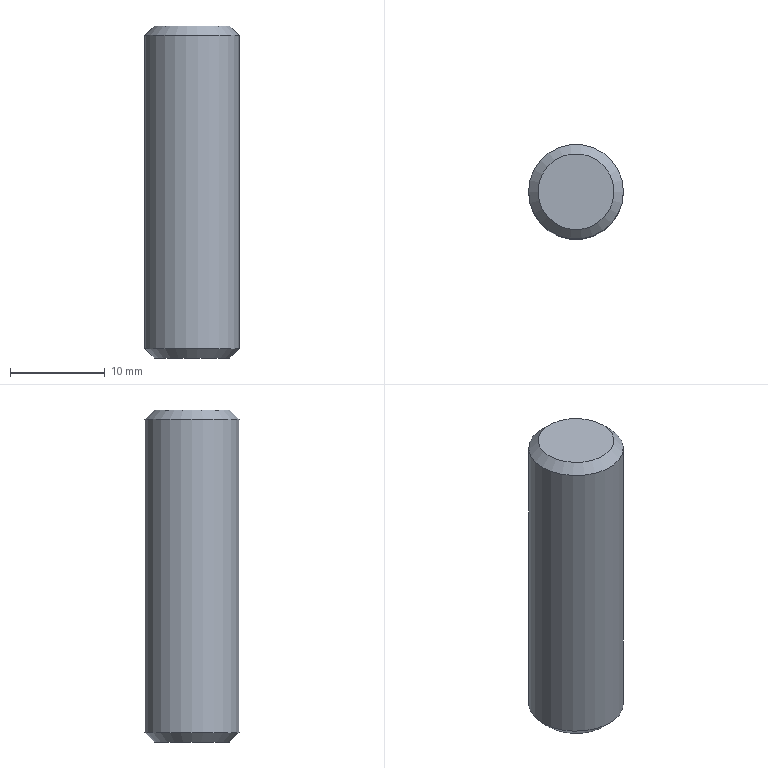Component | NX | EJECTOR_ROD | 1 solid | 5 faces | box 10 x 10 x 35 mm | volume 2720 mm3 | plane 2 | cone 2 | cylinder 1 | commonest cylinder face diameters 10 x1
STEP:
#1=CARTESIAN_POINT('',(0.,0.,0.));
#2=DIRECTION('',(0.,0.,1.));
#3=DIRECTION('',(1.,0.,0.));
#4=AXIS2_PLACEMENT_3D('',#1,#2,#3);
#5=CARTESIAN_POINT('',(24.,80.,198.));
#6=VERTEX_POINT('',#5);
#7=CARTESIAN_POINT('',(20.,80.,198.));
#8=DIRECTION('',(0.,0.,1.));
#9=DIRECTION('',(1.,0.,0.));
#10=AXIS2_PLACEMENT_3D('',#7,#8,#9);
#11=CIRCLE('',#10,4.);
#12=CARTESIAN_POINT('',(20.,80.,198.));
#13=DIRECTION('',(0.,0.,1.));
#14=DIRECTION('',(1.,0.,0.));
#15=AXIS2_PLACEMENT_3D('',#12,#13,#14);
#16=PLANE('',#15);
#17=CARTESIAN_POINT('',(0.,0.));
#18=DIRECTION('',(1.,0.));
#19=AXIS2_PLACEMENT_2D('',#17,#18);
#20=CIRCLE('',#19,4.);
#21=(GEOMETRIC_REPRESENTATION_CONTEXT(2)PARAMETRIC_REPRESENTATION_CONTEXT()REPRESENTATION_CONTEXT('',''));
#22=DEFINITIONAL_REPRESENTATION('',(#20),#21);
#23=PCURVE('',#16,#22);
#24=CARTESIAN_POINT('',(20.,80.,197.));
#25=DIRECTION('',(0.,0.,-1.));
#26=DIRECTION('',(-1.,0.,0.));
#27=AXIS2_PLACEMENT_3D('',#24,#25,#26);
#28=CONICAL_SURFACE('',#27,5.,0.7854);
#29=CARTESIAN_POINT('',(9.425,-1.));
#30=DIRECTION('',(-1.,0.));
#31=VECTOR('',#30,1.);
#32=LINE('',#29,#31);
#33=(GEOMETRIC_REPRESENTATION_CONTEXT(2)PARAMETRIC_REPRESENTATION_CONTEXT()REPRESENTATION_CONTEXT('',''));
#34=DEFINITIONAL_REPRESENTATION('',(#32),#33);
#35=PCURVE('',#28,#34);
#36=SURFACE_CURVE('',#11,(#23,#35),.PCURVE_S1.);
#37=EDGE_CURVE('',#6,#6,#36,.T.);
#38=ORIENTED_EDGE('',*,*,#37,.T.);
#39=EDGE_LOOP('',(#38));
#40=FACE_BOUND('',#39,.T.);
#41=ADVANCED_FACE('',(#40),#16,.T.);
#42=CARTESIAN_POINT('',(16.,80.,163.));
#43=VERTEX_POINT('',#42);
#44=CARTESIAN_POINT('',(20.,80.,163.));
#45=DIRECTION('',(0.,0.,-1.));
#46=DIRECTION('',(-1.,0.,0.));
#47=AXIS2_PLACEMENT_3D('',#44,#45,#46);
#48=CIRCLE('',#47,4.);
#49=CARTESIAN_POINT('',(20.,80.,163.));
#50=DIRECTION('',(0.,0.,-1.));
#51=DIRECTION('',(-1.,0.,0.));
#52=AXIS2_PLACEMENT_3D('',#49,#50,#51);
#53=PLANE('',#52);
#54=CARTESIAN_POINT('',(0.,0.));
#55=DIRECTION('',(1.,0.));
#56=AXIS2_PLACEMENT_2D('',#54,#55);
#57=CIRCLE('',#56,4.);
#58=(GEOMETRIC_REPRESENTATION_CONTEXT(2)PARAMETRIC_REPRESENTATION_CONTEXT()REPRESENTATION_CONTEXT('',''));
#59=DEFINITIONAL_REPRESENTATION('',(#57),#58);
#60=PCURVE('',#53,#59);
#61=CARTESIAN_POINT('',(20.,80.,164.));
#62=DIRECTION('',(0.,0.,1.));
#63=DIRECTION('',(1.,0.,0.));
#64=AXIS2_PLACEMENT_3D('',#61,#62,#63);
#65=CONICAL_SURFACE('',#64,5.,0.7854);
#66=CARTESIAN_POINT('',(9.425,-1.));
#67=DIRECTION('',(-1.,0.));
#68=VECTOR('',#67,1.);
#69=LINE('',#66,#68);
#70=(GEOMETRIC_REPRESENTATION_CONTEXT(2)PARAMETRIC_REPRESENTATION_CONTEXT()REPRESENTATION_CONTEXT('',''));
#71=DEFINITIONAL_REPRESENTATION('',(#69),#70);
#72=PCURVE('',#65,#71);
#73=SURFACE_CURVE('',#48,(#60,#72),.PCURVE_S1.);
#74=EDGE_CURVE('',#43,#43,#73,.T.);
#75=ORIENTED_EDGE('',*,*,#74,.T.);
#76=EDGE_LOOP('',(#75));
#77=FACE_BOUND('',#76,.T.);
#78=ADVANCED_FACE('',(#77),#53,.T.);
#79=CARTESIAN_POINT('',(15.,80.,164.));
#80=VERTEX_POINT('',#79);
#81=CARTESIAN_POINT('',(25.,80.,164.));
#82=VERTEX_POINT('',#81);
#83=CARTESIAN_POINT('',(20.,80.,164.));
#84=DIRECTION('',(0.,0.,1.));
#85=DIRECTION('',(-1.,0.,0.));
#86=AXIS2_PLACEMENT_3D('',#83,#84,#85);
#87=CIRCLE('',#86,5.);
#88=CARTESIAN_POINT('',(20.,80.,163.));
#89=DIRECTION('',(0.,0.,1.));
#90=DIRECTION('',(1.,0.,0.));
#91=AXIS2_PLACEMENT_3D('',#88,#89,#90);
#92=CYLINDRICAL_SURFACE('',#91,5.);
#93=CARTESIAN_POINT('',(3.142,1.));
#94=DIRECTION('',(1.,0.));
#95=VECTOR('',#94,1.);
#96=LINE('',#93,#95);
#97=(GEOMETRIC_REPRESENTATION_CONTEXT(2)PARAMETRIC_REPRESENTATION_CONTEXT()REPRESENTATION_CONTEXT('',''));
#98=DEFINITIONAL_REPRESENTATION('',(#96),#97);
#99=PCURVE('',#92,#98);
#100=CARTESIAN_POINT('',(3.142,0.));
#101=DIRECTION('',(1.,0.));
#102=VECTOR('',#101,1.);
#103=LINE('',#100,#102);
#104=(GEOMETRIC_REPRESENTATION_CONTEXT(2)PARAMETRIC_REPRESENTATION_CONTEXT()REPRESENTATION_CONTEXT('',''));
#105=DEFINITIONAL_REPRESENTATION('',(#103),#104);
#106=PCURVE('',#65,#105);
#107=SURFACE_CURVE('',#87,(#99,#106),.PCURVE_S1.);
#108=EDGE_CURVE('',#80,#82,#107,.T.);
#109=ORIENTED_EDGE('',*,*,#108,.T.);
#110=CARTESIAN_POINT('',(25.,80.,197.));
#111=VERTEX_POINT('',#110);
#112=CARTESIAN_POINT('',(25.,80.,164.));
#113=CARTESIAN_POINT('',(25.,80.,197.));
#114=B_SPLINE_CURVE_WITH_KNOTS('',1,(#112,#113),.UNSPECIFIED.,.F.,.F.,(2,2),(1.,34.),.PIECEWISE_BEZIER_KNOTS.);
#115=CARTESIAN_POINT('',(6.283,0.));
#116=DIRECTION('',(0.,1.));
#117=VECTOR('',#116,1.);
#118=LINE('',#115,#117);
#119=(GEOMETRIC_REPRESENTATION_CONTEXT(2)PARAMETRIC_REPRESENTATION_CONTEXT()REPRESENTATION_CONTEXT('',''));
#120=DEFINITIONAL_REPRESENTATION('',(#118),#119);
#121=PCURVE('',#92,#120);
#122=CARTESIAN_POINT('',(0.,0.));
#123=DIRECTION('',(0.,1.));
#124=VECTOR('',#123,1.);
#125=LINE('',#122,#124);
#126=(GEOMETRIC_REPRESENTATION_CONTEXT(2)PARAMETRIC_REPRESENTATION_CONTEXT()REPRESENTATION_CONTEXT('',''));
#127=DEFINITIONAL_REPRESENTATION('',(#125),#126);
#128=PCURVE('',#92,#127);
#129=SEAM_CURVE('',#114,(#121,#128),.PCURVE_S1.);
#130=EDGE_CURVE('',#82,#111,#129,.T.);
#131=ORIENTED_EDGE('',*,*,#130,.T.);
#132=CARTESIAN_POINT('',(20.,80.,197.));
#133=DIRECTION('',(0.,0.,-1.));
#134=DIRECTION('',(1.,0.,0.));
#135=AXIS2_PLACEMENT_3D('',#132,#133,#134);
#136=CIRCLE('',#135,5.);
#137=CARTESIAN_POINT('',(6.283,34.));
#138=DIRECTION('',(-1.,0.));
#139=VECTOR('',#138,1.);
#140=LINE('',#137,#139);
#141=(GEOMETRIC_REPRESENTATION_CONTEXT(2)PARAMETRIC_REPRESENTATION_CONTEXT()REPRESENTATION_CONTEXT('',''));
#142=DEFINITIONAL_REPRESENTATION('',(#140),#141);
#143=PCURVE('',#92,#142);
#144=CARTESIAN_POINT('',(3.142,0.));
#145=DIRECTION('',(1.,0.));
#146=VECTOR('',#145,1.);
#147=LINE('',#144,#146);
#148=(GEOMETRIC_REPRESENTATION_CONTEXT(2)PARAMETRIC_REPRESENTATION_CONTEXT()REPRESENTATION_CONTEXT('',''));
#149=DEFINITIONAL_REPRESENTATION('',(#147),#148);
#150=PCURVE('',#28,#149);
#151=SURFACE_CURVE('',#136,(#143,#150),.PCURVE_S1.);
#152=EDGE_CURVE('',#111,#111,#151,.T.);
#153=ORIENTED_EDGE('',*,*,#152,.T.);
#154=ORIENTED_EDGE('',*,*,#130,.F.);
#155=CARTESIAN_POINT('',(20.,80.,164.));
#156=DIRECTION('',(0.,0.,1.));
#157=DIRECTION('',(-1.,0.,0.));
#158=AXIS2_PLACEMENT_3D('',#155,#156,#157);
#159=CIRCLE('',#158,5.);
#160=CARTESIAN_POINT('',(-3.142,1.));
#161=DIRECTION('',(1.,0.));
#162=VECTOR('',#161,1.);
#163=LINE('',#160,#162);
#164=(GEOMETRIC_REPRESENTATION_CONTEXT(2)PARAMETRIC_REPRESENTATION_CONTEXT()REPRESENTATION_CONTEXT('',''));
#165=DEFINITIONAL_REPRESENTATION('',(#163),#164);
#166=PCURVE('',#92,#165);
#167=CARTESIAN_POINT('',(3.142,0.));
#168=DIRECTION('',(1.,0.));
#169=VECTOR('',#168,1.);
#170=LINE('',#167,#169);
#171=(GEOMETRIC_REPRESENTATION_CONTEXT(2)PARAMETRIC_REPRESENTATION_CONTEXT()REPRESENTATION_CONTEXT('',''));
#172=DEFINITIONAL_REPRESENTATION('',(#170),#171);
#173=PCURVE('',#65,#172);
#174=SURFACE_CURVE('',#159,(#166,#173),.PCURVE_S1.);
#175=EDGE_CURVE('',#82,#80,#174,.T.);
#176=ORIENTED_EDGE('',*,*,#175,.T.);
#177=EDGE_LOOP('',(#109,#131,#153,#154,#176));
#178=FACE_BOUND('',#177,.T.);
#179=ADVANCED_FACE('',(#178),#92,.T.);
#180=ORIENTED_EDGE('',*,*,#74,.F.);
#181=CARTESIAN_POINT('',(16.,80.,163.));
#182=CARTESIAN_POINT('',(15.,80.,164.));
#183=B_SPLINE_CURVE_WITH_KNOTS('',1,(#181,#182),.UNSPECIFIED.,.F.,.F.,(2,2),(-1.414,0.),.PIECEWISE_BEZIER_KNOTS.);
#184=CARTESIAN_POINT('',(9.425,0.));
#185=DIRECTION('',(0.,1.));
#186=VECTOR('',#185,1.);
#187=LINE('',#184,#186);
#188=(GEOMETRIC_REPRESENTATION_CONTEXT(2)PARAMETRIC_REPRESENTATION_CONTEXT()REPRESENTATION_CONTEXT('',''));
#189=DEFINITIONAL_REPRESENTATION('',(#187),#188);
#190=PCURVE('',#65,#189);
#191=CARTESIAN_POINT('',(3.142,0.));
#192=DIRECTION('',(0.,1.));
#193=VECTOR('',#192,1.);
#194=LINE('',#191,#193);
#195=(GEOMETRIC_REPRESENTATION_CONTEXT(2)PARAMETRIC_REPRESENTATION_CONTEXT()REPRESENTATION_CONTEXT('',''));
#196=DEFINITIONAL_REPRESENTATION('',(#194),#195);
#197=PCURVE('',#65,#196);
#198=SEAM_CURVE('',#183,(#190,#197),.PCURVE_S1.);
#199=EDGE_CURVE('',#43,#80,#198,.T.);
#200=ORIENTED_EDGE('',*,*,#199,.T.);
#201=ORIENTED_EDGE('',*,*,#175,.F.);
#202=ORIENTED_EDGE('',*,*,#108,.F.);
#203=ORIENTED_EDGE('',*,*,#199,.F.);
#204=EDGE_LOOP('',(#180,#200,#201,#202,#203));
#205=FACE_BOUND('',#204,.T.);
#206=ADVANCED_FACE('',(#205),#65,.T.);
#207=ORIENTED_EDGE('',*,*,#37,.F.);
#208=CARTESIAN_POINT('',(24.,80.,198.));
#209=CARTESIAN_POINT('',(25.,80.,197.));
#210=B_SPLINE_CURVE_WITH_KNOTS('',1,(#208,#209),.UNSPECIFIED.,.F.,.F.,(2,2),(-1.414,0.),.PIECEWISE_BEZIER_KNOTS.);
#211=CARTESIAN_POINT('',(9.425,0.));
#212=DIRECTION('',(0.,1.));
#213=VECTOR('',#212,1.);
#214=LINE('',#211,#213);
#215=(GEOMETRIC_REPRESENTATION_CONTEXT(2)PARAMETRIC_REPRESENTATION_CONTEXT()REPRESENTATION_CONTEXT('',''));
#216=DEFINITIONAL_REPRESENTATION('',(#214),#215);
#217=PCURVE('',#28,#216);
#218=CARTESIAN_POINT('',(3.142,0.));
#219=DIRECTION('',(0.,1.));
#220=VECTOR('',#219,1.);
#221=LINE('',#218,#220);
#222=(GEOMETRIC_REPRESENTATION_CONTEXT(2)PARAMETRIC_REPRESENTATION_CONTEXT()REPRESENTATION_CONTEXT('',''));
#223=DEFINITIONAL_REPRESENTATION('',(#221),#222);
#224=PCURVE('',#28,#223);
#225=SEAM_CURVE('',#210,(#217,#224),.PCURVE_S1.);
#226=EDGE_CURVE('',#6,#111,#225,.T.);
#227=ORIENTED_EDGE('',*,*,#226,.T.);
#228=ORIENTED_EDGE('',*,*,#152,.F.);
#229=ORIENTED_EDGE('',*,*,#226,.F.);
#230=EDGE_LOOP('',(#207,#227,#228,#229));
#231=FACE_BOUND('',#230,.T.);
#232=ADVANCED_FACE('',(#231),#28,.T.);
#233=CLOSED_SHELL('',(#41,#78,#179,#206,#232));
#234=MANIFOLD_SOLID_BREP('',#233);
#235=(LENGTH_UNIT()NAMED_UNIT(*)SI_UNIT(.MILLI.,.METRE.));
#236=UNCERTAINTY_MEASURE_WITH_UNIT(LENGTH_MEASURE(0.00001),#235,'','');
#237=(NAMED_UNIT(*)PLANE_ANGLE_UNIT()SI_UNIT($,.RADIAN.));
#238=(NAMED_UNIT(*)SI_UNIT($,.STERADIAN.)SOLID_ANGLE_UNIT());
#239=(GEOMETRIC_REPRESENTATION_CONTEXT(3)GLOBAL_UNCERTAINTY_ASSIGNED_CONTEXT((#236))GLOBAL_UNIT_ASSIGNED_CONTEXT((#235,#237,#238))REPRESENTATION_CONTEXT('',''));
#240=ADVANCED_BREP_SHAPE_REPRESENTATION('',(#4,#234),#239);